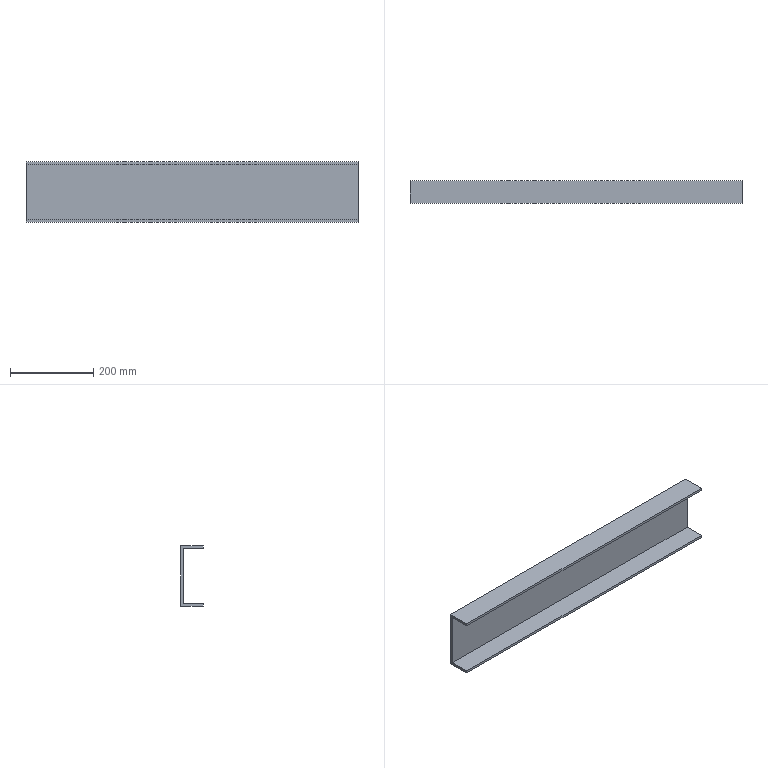Component | SolidWorks | JF21-80.1-1-3(_)-1-SOLID52-1 | 1 solid | 10 faces | box 800 x 55 x 145 mm | volume 1166400 mm3 | plane 10
STEP:
#1=COLOUR_RGB('',0.7922,0.8196,0.9333);
#2=FILL_AREA_STYLE_COLOUR('',#1);
#3=FILL_AREA_STYLE('',(#2));
#4=SURFACE_STYLE_FILL_AREA(#3);
#5=SURFACE_SIDE_STYLE('',(#4));
#6=SURFACE_STYLE_USAGE(.BOTH.,#5);
#7=PRESENTATION_STYLE_ASSIGNMENT((#6));
#8=CARTESIAN_POINT('',(15.748,-86.417,50.591));
#9=VERTEX_POINT('',#8);
#10=CARTESIAN_POINT('',(15.748,-88.583,50.591));
#11=VERTEX_POINT('',#10);
#12=CARTESIAN_POINT('',(15.748,-88.583,50.591));
#13=DIRECTION('',(0.,-1.,0.));
#14=VECTOR('',#13,39.37);
#15=LINE('',#12,#14);
#16=EDGE_CURVE('',#9,#11,#15,.T.);
#17=ORIENTED_EDGE('',*,*,#16,.F.);
#18=CARTESIAN_POINT('',(-15.748,-86.417,50.591));
#19=VERTEX_POINT('',#18);
#20=CARTESIAN_POINT('',(21.854,-86.417,50.591));
#21=DIRECTION('',(-1.,0.,0.));
#22=VECTOR('',#21,39.37);
#23=LINE('',#20,#22);
#24=EDGE_CURVE('',#9,#19,#23,.T.);
#25=ORIENTED_EDGE('',*,*,#24,.T.);
#26=CARTESIAN_POINT('',(-15.748,-88.583,50.591));
#27=VERTEX_POINT('',#26);
#28=CARTESIAN_POINT('',(-15.748,-88.583,50.591));
#29=DIRECTION('',(0.,-1.,0.));
#30=VECTOR('',#29,39.37);
#31=LINE('',#28,#30);
#32=EDGE_CURVE('',#19,#27,#31,.T.);
#33=ORIENTED_EDGE('',*,*,#32,.T.);
#34=CARTESIAN_POINT('',(21.854,-88.583,50.591));
#35=DIRECTION('',(-1.,0.,0.));
#36=VECTOR('',#35,39.37);
#37=LINE('',#34,#36);
#38=EDGE_CURVE('',#11,#27,#37,.T.);
#39=ORIENTED_EDGE('',*,*,#38,.F.);
#40=EDGE_LOOP('',(#17,#25,#33,#39));
#41=FACE_OUTER_BOUND('',#40,.T.);
#42=CARTESIAN_POINT('',(21.854,-88.583,50.591));
#43=DIRECTION('',(0.,0.,-1.));
#44=DIRECTION('',(1.,0.,0.));
#45=AXIS2_PLACEMENT_3D('',#42,#43,#44);
#46=PLANE('',#45);
#47=ADVANCED_FACE('',(#41),#46,.F.);
#48=CARTESIAN_POINT('',(15.748,-88.583,50.354));
#49=VERTEX_POINT('',#48);
#50=CARTESIAN_POINT('',(15.748,-88.583,50.591));
#51=DIRECTION('',(0.,0.,-1.));
#52=VECTOR('',#51,39.37);
#53=LINE('',#50,#52);
#54=EDGE_CURVE('',#11,#49,#53,.T.);
#55=ORIENTED_EDGE('',*,*,#54,.F.);
#56=ORIENTED_EDGE('',*,*,#38,.T.);
#57=CARTESIAN_POINT('',(-15.748,-88.583,50.354));
#58=VERTEX_POINT('',#57);
#59=CARTESIAN_POINT('',(-15.748,-88.583,50.591));
#60=DIRECTION('',(0.,0.,-1.));
#61=VECTOR('',#60,39.37);
#62=LINE('',#59,#61);
#63=EDGE_CURVE('',#27,#58,#62,.T.);
#64=ORIENTED_EDGE('',*,*,#63,.T.);
#65=CARTESIAN_POINT('',(21.854,-88.583,50.354));
#66=DIRECTION('',(-1.,0.,0.));
#67=VECTOR('',#66,39.37);
#68=LINE('',#65,#67);
#69=EDGE_CURVE('',#49,#58,#68,.T.);
#70=ORIENTED_EDGE('',*,*,#69,.F.);
#71=EDGE_LOOP('',(#55,#56,#64,#70));
#72=FACE_OUTER_BOUND('',#71,.T.);
#73=CARTESIAN_POINT('',(21.854,-88.583,50.591));
#74=DIRECTION('',(0.,1.,0.));
#75=DIRECTION('',(0.,0.,-1.));
#76=AXIS2_PLACEMENT_3D('',#73,#74,#75);
#77=PLANE('',#76);
#78=ADVANCED_FACE('',(#72),#77,.F.);
#79=CARTESIAN_POINT('',(15.748,-86.654,50.354));
#80=VERTEX_POINT('',#79);
#81=CARTESIAN_POINT('',(15.748,-88.583,50.354));
#82=DIRECTION('',(0.,1.,0.));
#83=VECTOR('',#82,39.37);
#84=LINE('',#81,#83);
#85=EDGE_CURVE('',#49,#80,#84,.T.);
#86=ORIENTED_EDGE('',*,*,#85,.F.);
#87=ORIENTED_EDGE('',*,*,#69,.T.);
#88=CARTESIAN_POINT('',(-15.748,-86.654,50.354));
#89=VERTEX_POINT('',#88);
#90=CARTESIAN_POINT('',(-15.748,-88.583,50.354));
#91=DIRECTION('',(0.,1.,0.));
#92=VECTOR('',#91,39.37);
#93=LINE('',#90,#92);
#94=EDGE_CURVE('',#58,#89,#93,.T.);
#95=ORIENTED_EDGE('',*,*,#94,.T.);
#96=CARTESIAN_POINT('',(21.854,-86.654,50.354));
#97=DIRECTION('',(-1.,0.,0.));
#98=VECTOR('',#97,39.37);
#99=LINE('',#96,#98);
#100=EDGE_CURVE('',#80,#89,#99,.T.);
#101=ORIENTED_EDGE('',*,*,#100,.F.);
#102=EDGE_LOOP('',(#86,#87,#95,#101));
#103=FACE_OUTER_BOUND('',#102,.T.);
#104=CARTESIAN_POINT('',(21.854,-88.583,50.354));
#105=DIRECTION('',(0.,0.,1.));
#106=DIRECTION('',(-1.,0.,0.));
#107=AXIS2_PLACEMENT_3D('',#104,#105,#106);
#108=PLANE('',#107);
#109=ADVANCED_FACE('',(#103),#108,.F.);
#110=CARTESIAN_POINT('',(15.748,-86.654,45.118));
#111=VERTEX_POINT('',#110);
#112=CARTESIAN_POINT('',(15.748,-86.654,50.354));
#113=DIRECTION('',(0.,0.,-1.));
#114=VECTOR('',#113,39.37);
#115=LINE('',#112,#114);
#116=EDGE_CURVE('',#80,#111,#115,.T.);
#117=ORIENTED_EDGE('',*,*,#116,.F.);
#118=ORIENTED_EDGE('',*,*,#100,.T.);
#119=CARTESIAN_POINT('',(-15.748,-86.654,45.118));
#120=VERTEX_POINT('',#119);
#121=CARTESIAN_POINT('',(-15.748,-86.654,50.354));
#122=DIRECTION('',(0.,0.,-1.));
#123=VECTOR('',#122,39.37);
#124=LINE('',#121,#123);
#125=EDGE_CURVE('',#89,#120,#124,.T.);
#126=ORIENTED_EDGE('',*,*,#125,.T.);
#127=CARTESIAN_POINT('',(21.854,-86.654,45.118));
#128=DIRECTION('',(-1.,0.,0.));
#129=VECTOR('',#128,39.37);
#130=LINE('',#127,#129);
#131=EDGE_CURVE('',#111,#120,#130,.T.);
#132=ORIENTED_EDGE('',*,*,#131,.F.);
#133=EDGE_LOOP('',(#117,#118,#126,#132));
#134=FACE_OUTER_BOUND('',#133,.T.);
#135=CARTESIAN_POINT('',(21.854,-86.654,50.354));
#136=DIRECTION('',(0.,1.,0.));
#137=DIRECTION('',(0.,0.,-1.));
#138=AXIS2_PLACEMENT_3D('',#135,#136,#137);
#139=PLANE('',#138);
#140=ADVANCED_FACE('',(#134),#139,.F.);
#141=CARTESIAN_POINT('',(15.748,-88.583,45.118));
#142=VERTEX_POINT('',#141);
#143=CARTESIAN_POINT('',(15.748,-86.654,45.118));
#144=DIRECTION('',(0.,-1.,0.));
#145=VECTOR('',#144,39.37);
#146=LINE('',#143,#145);
#147=EDGE_CURVE('',#111,#142,#146,.T.);
#148=ORIENTED_EDGE('',*,*,#147,.F.);
#149=ORIENTED_EDGE('',*,*,#131,.T.);
#150=CARTESIAN_POINT('',(-15.748,-88.583,45.118));
#151=VERTEX_POINT('',#150);
#152=CARTESIAN_POINT('',(-15.748,-86.654,45.118));
#153=DIRECTION('',(0.,-1.,0.));
#154=VECTOR('',#153,39.37);
#155=LINE('',#152,#154);
#156=EDGE_CURVE('',#120,#151,#155,.T.);
#157=ORIENTED_EDGE('',*,*,#156,.T.);
#158=CARTESIAN_POINT('',(21.854,-88.583,45.118));
#159=DIRECTION('',(-1.,0.,0.));
#160=VECTOR('',#159,39.37);
#161=LINE('',#158,#160);
#162=EDGE_CURVE('',#142,#151,#161,.T.);
#163=ORIENTED_EDGE('',*,*,#162,.F.);
#164=EDGE_LOOP('',(#148,#149,#157,#163));
#165=FACE_OUTER_BOUND('',#164,.T.);
#166=CARTESIAN_POINT('',(21.854,-86.654,45.118));
#167=DIRECTION('',(0.,0.,-1.));
#168=DIRECTION('',(1.,0.,0.));
#169=AXIS2_PLACEMENT_3D('',#166,#167,#168);
#170=PLANE('',#169);
#171=ADVANCED_FACE('',(#165),#170,.F.);
#172=CARTESIAN_POINT('',(15.748,-88.583,44.882));
#173=VERTEX_POINT('',#172);
#174=CARTESIAN_POINT('',(15.748,-88.583,45.118));
#175=DIRECTION('',(0.,0.,-1.));
#176=VECTOR('',#175,39.37);
#177=LINE('',#174,#176);
#178=EDGE_CURVE('',#142,#173,#177,.T.);
#179=ORIENTED_EDGE('',*,*,#178,.F.);
#180=ORIENTED_EDGE('',*,*,#162,.T.);
#181=CARTESIAN_POINT('',(-15.748,-88.583,44.882));
#182=VERTEX_POINT('',#181);
#183=CARTESIAN_POINT('',(-15.748,-88.583,45.118));
#184=DIRECTION('',(0.,0.,-1.));
#185=VECTOR('',#184,39.37);
#186=LINE('',#183,#185);
#187=EDGE_CURVE('',#151,#182,#186,.T.);
#188=ORIENTED_EDGE('',*,*,#187,.T.);
#189=CARTESIAN_POINT('',(21.854,-88.583,44.882));
#190=DIRECTION('',(-1.,0.,0.));
#191=VECTOR('',#190,39.37);
#192=LINE('',#189,#191);
#193=EDGE_CURVE('',#173,#182,#192,.T.);
#194=ORIENTED_EDGE('',*,*,#193,.F.);
#195=EDGE_LOOP('',(#179,#180,#188,#194));
#196=FACE_OUTER_BOUND('',#195,.T.);
#197=CARTESIAN_POINT('',(21.854,-88.583,45.118));
#198=DIRECTION('',(0.,1.,0.));
#199=DIRECTION('',(0.,0.,-1.));
#200=AXIS2_PLACEMENT_3D('',#197,#198,#199);
#201=PLANE('',#200);
#202=ADVANCED_FACE('',(#196),#201,.F.);
#203=CARTESIAN_POINT('',(15.748,-86.417,44.882));
#204=VERTEX_POINT('',#203);
#205=CARTESIAN_POINT('',(15.748,-88.583,44.882));
#206=DIRECTION('',(0.,1.,0.));
#207=VECTOR('',#206,39.37);
#208=LINE('',#205,#207);
#209=EDGE_CURVE('',#173,#204,#208,.T.);
#210=ORIENTED_EDGE('',*,*,#209,.F.);
#211=ORIENTED_EDGE('',*,*,#193,.T.);
#212=CARTESIAN_POINT('',(-15.748,-86.417,44.882));
#213=VERTEX_POINT('',#212);
#214=CARTESIAN_POINT('',(-15.748,-88.583,44.882));
#215=DIRECTION('',(0.,1.,0.));
#216=VECTOR('',#215,39.37);
#217=LINE('',#214,#216);
#218=EDGE_CURVE('',#182,#213,#217,.T.);
#219=ORIENTED_EDGE('',*,*,#218,.T.);
#220=CARTESIAN_POINT('',(21.854,-86.417,44.882));
#221=DIRECTION('',(-1.,0.,0.));
#222=VECTOR('',#221,39.37);
#223=LINE('',#220,#222);
#224=EDGE_CURVE('',#204,#213,#223,.T.);
#225=ORIENTED_EDGE('',*,*,#224,.F.);
#226=EDGE_LOOP('',(#210,#211,#219,#225));
#227=FACE_OUTER_BOUND('',#226,.T.);
#228=CARTESIAN_POINT('',(21.854,-88.583,44.882));
#229=DIRECTION('',(0.,0.,1.));
#230=DIRECTION('',(-1.,0.,0.));
#231=AXIS2_PLACEMENT_3D('',#228,#229,#230);
#232=PLANE('',#231);
#233=ADVANCED_FACE('',(#227),#232,.F.);
#234=CARTESIAN_POINT('',(15.748,-86.417,50.591));
#235=DIRECTION('',(0.,0.,1.));
#236=VECTOR('',#235,39.37);
#237=LINE('',#234,#236);
#238=EDGE_CURVE('',#204,#9,#237,.T.);
#239=ORIENTED_EDGE('',*,*,#238,.F.);
#240=ORIENTED_EDGE('',*,*,#224,.T.);
#241=CARTESIAN_POINT('',(-15.748,-86.417,50.591));
#242=DIRECTION('',(0.,0.,1.));
#243=VECTOR('',#242,39.37);
#244=LINE('',#241,#243);
#245=EDGE_CURVE('',#213,#19,#244,.T.);
#246=ORIENTED_EDGE('',*,*,#245,.T.);
#247=ORIENTED_EDGE('',*,*,#24,.F.);
#248=EDGE_LOOP('',(#239,#240,#246,#247));
#249=FACE_OUTER_BOUND('',#248,.T.);
#250=CARTESIAN_POINT('',(21.854,-86.417,50.591));
#251=DIRECTION('',(0.,-1.,0.));
#252=DIRECTION('',(0.,0.,1.));
#253=AXIS2_PLACEMENT_3D('',#250,#251,#252);
#254=PLANE('',#253);
#255=ADVANCED_FACE('',(#249),#254,.F.);
#256=ORIENTED_EDGE('',*,*,#32,.F.);
#257=ORIENTED_EDGE('',*,*,#245,.F.);
#258=ORIENTED_EDGE('',*,*,#218,.F.);
#259=ORIENTED_EDGE('',*,*,#187,.F.);
#260=ORIENTED_EDGE('',*,*,#156,.F.);
#261=ORIENTED_EDGE('',*,*,#125,.F.);
#262=ORIENTED_EDGE('',*,*,#94,.F.);
#263=ORIENTED_EDGE('',*,*,#63,.F.);
#264=EDGE_LOOP('',(#256,#257,#258,#259,#260,#261,#262,#263));
#265=FACE_OUTER_BOUND('',#264,.T.);
#266=CARTESIAN_POINT('',(-15.748,-86.417,50.591));
#267=DIRECTION('',(-1.,0.,0.));
#268=DIRECTION('',(0.,0.,-1.));
#269=AXIS2_PLACEMENT_3D('',#266,#267,#268);
#270=PLANE('',#269);
#271=ADVANCED_FACE('',(#265),#270,.T.);
#272=ORIENTED_EDGE('',*,*,#238,.T.);
#273=ORIENTED_EDGE('',*,*,#16,.T.);
#274=ORIENTED_EDGE('',*,*,#54,.T.);
#275=ORIENTED_EDGE('',*,*,#85,.T.);
#276=ORIENTED_EDGE('',*,*,#116,.T.);
#277=ORIENTED_EDGE('',*,*,#147,.T.);
#278=ORIENTED_EDGE('',*,*,#178,.T.);
#279=ORIENTED_EDGE('',*,*,#209,.T.);
#280=EDGE_LOOP('',(#272,#273,#274,#275,#276,#277,#278,#279));
#281=FACE_OUTER_BOUND('',#280,.T.);
#282=CARTESIAN_POINT('',(15.748,-10.551,2.638));
#283=DIRECTION('',(1.,0.,0.));
#284=DIRECTION('',(0.,0.,1.));
#285=AXIS2_PLACEMENT_3D('',#282,#283,#284);
#286=PLANE('',#285);
#287=ADVANCED_FACE('',(#281),#286,.T.);
#288=CLOSED_SHELL('',(#47,#78,#109,#140,#171,#202,#233,#255,#271,#287));
#289=MANIFOLD_SOLID_BREP('',#288);
#290=STYLED_ITEM('',(#7),#289);
#291=PRESENTATION_LAYER_ASSIGNMENT('','',(#290));
#292=(LENGTH_UNIT()NAMED_UNIT(*)SI_UNIT($,.METRE.));
#293=LENGTH_MEASURE_WITH_UNIT(LENGTH_MEASURE(0.0254),#292);
#294=DIMENSIONAL_EXPONENTS(1.,0.,0.,0.,0.,0.,0.);
#295=(CONVERSION_BASED_UNIT('',#293)LENGTH_UNIT()NAMED_UNIT(#294));
#296=UNCERTAINTY_MEASURE_WITH_UNIT(LENGTH_MEASURE(0.00001),#295,'','');
#297=(NAMED_UNIT(*)PLANE_ANGLE_UNIT()SI_UNIT($,.RADIAN.));
#298=(NAMED_UNIT(*)SI_UNIT($,.STERADIAN.)SOLID_ANGLE_UNIT());
#299=(GEOMETRIC_REPRESENTATION_CONTEXT(3)GLOBAL_UNCERTAINTY_ASSIGNED_CONTEXT((#296))GLOBAL_UNIT_ASSIGNED_CONTEXT((#295,#297,#298))REPRESENTATION_CONTEXT('',''));
#300=MECHANICAL_DESIGN_GEOMETRIC_PRESENTATION_REPRESENTATION('',(#290),#299);
#301=CARTESIAN_POINT('',(0.,0.,0.));
#302=DIRECTION('',(0.,0.,1.));
#303=DIRECTION('',(1.,0.,0.));
#304=AXIS2_PLACEMENT_3D('',#301,#302,#303);
#305=(LENGTH_UNIT()NAMED_UNIT(*)SI_UNIT($,.METRE.));
#306=LENGTH_MEASURE_WITH_UNIT(LENGTH_MEASURE(0.0254),#305);
#307=DIMENSIONAL_EXPONENTS(1.,0.,0.,0.,0.,0.,0.);
#308=(CONVERSION_BASED_UNIT('',#306)LENGTH_UNIT()NAMED_UNIT(#307));
#309=UNCERTAINTY_MEASURE_WITH_UNIT(LENGTH_MEASURE(0.00001),#308,'','');
#310=(NAMED_UNIT(*)PLANE_ANGLE_UNIT()SI_UNIT($,.RADIAN.));
#311=(NAMED_UNIT(*)SI_UNIT($,.STERADIAN.)SOLID_ANGLE_UNIT());
#312=(GEOMETRIC_REPRESENTATION_CONTEXT(3)GLOBAL_UNCERTAINTY_ASSIGNED_CONTEXT((#309))GLOBAL_UNIT_ASSIGNED_CONTEXT((#308,#310,#311))REPRESENTATION_CONTEXT('',''));
#313=ADVANCED_BREP_SHAPE_REPRESENTATION('',(#289,#304),#312);